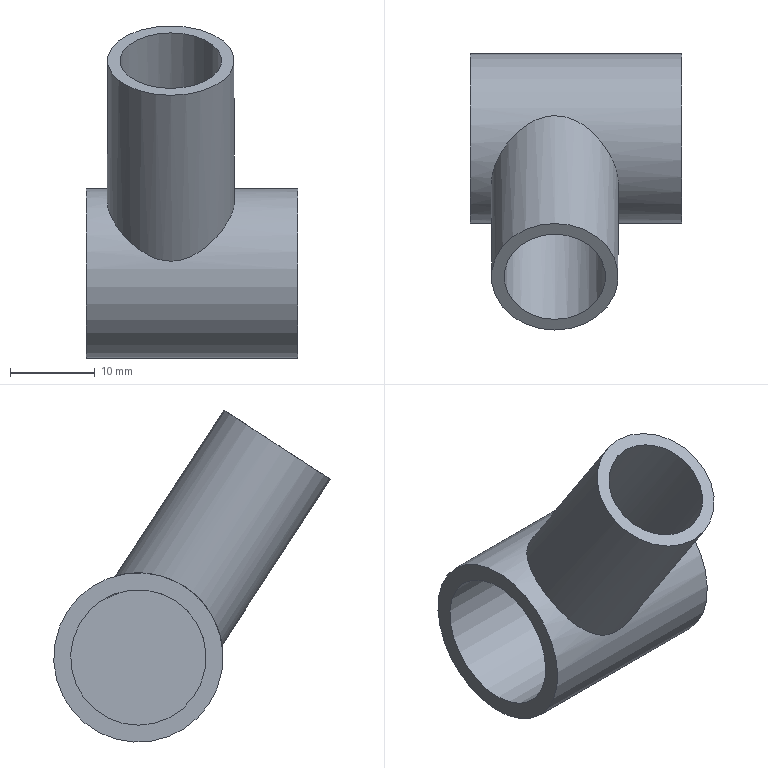Component | NX | CAP_3 | 1 solid | 8 faces | volume 4945 mm3 | cylinder 4 | plane 4 | commonest cylinder face diameters 20 x1 15 x1 16 x1 12 x1